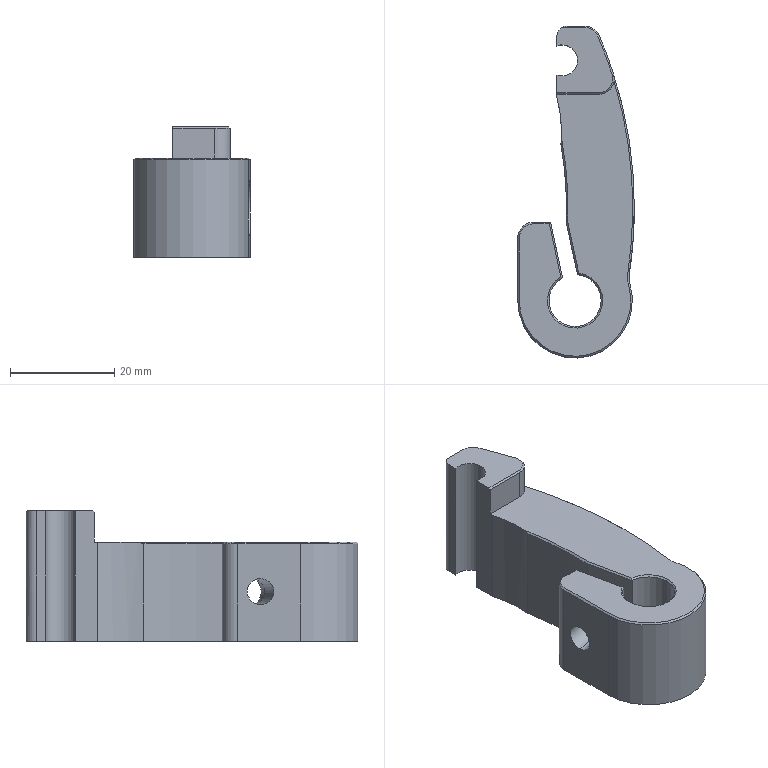CAM job | Mastercam | mm | 5 operations | part box 26.66 x 63.6 x 25
1. 2D High Speed (2D Area Mill) | 6 - 6 平铣刀
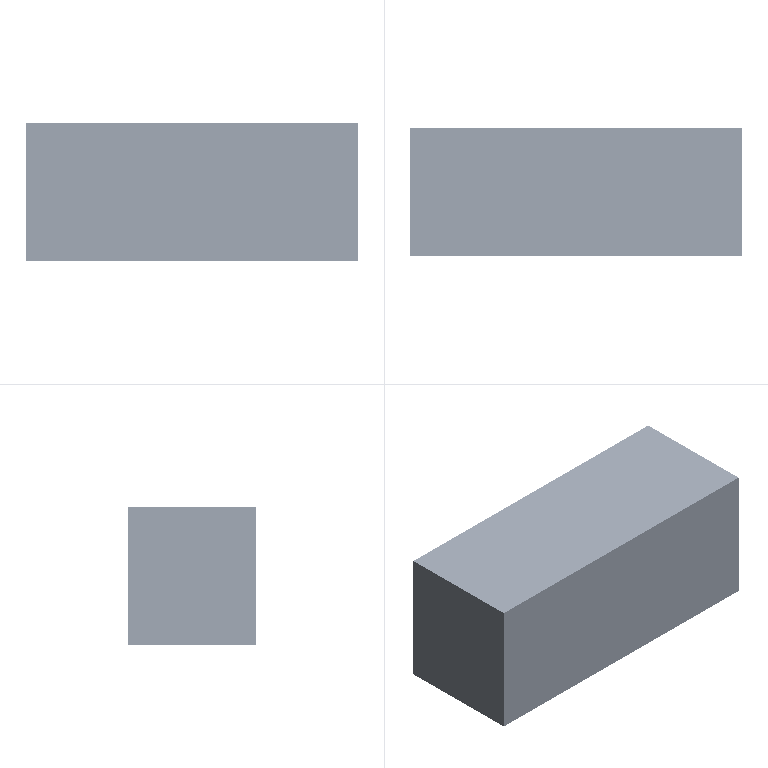2. Contour (2D) | 6 - 6 平铣刀
3. Contour (2D chamfer) | 7 - 6 倒角刀
4. Contour (Ramp) | 4 - 4 平铣刀
5. Contour (2D) | 4 - 4 平铣刀